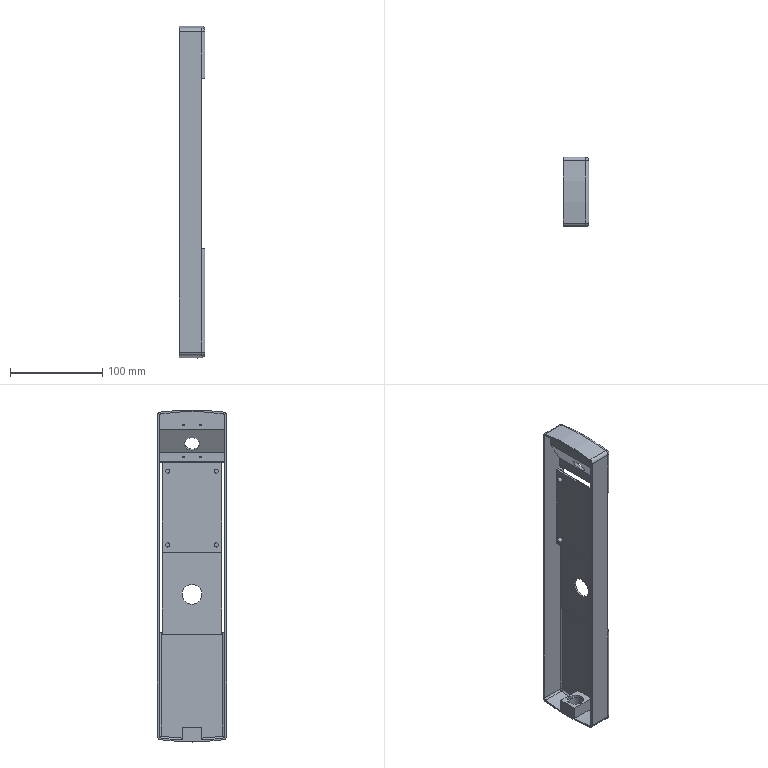Component | NX | TOUCH_HOUSING | 1 solid | 127 faces | volume 107924 mm3 | plane 60 | cylinder 50 | torus 9 | sphere 8 | commonest cylinder face diameters 4 x12 8 x8 1.6 x8 467.75 x4 4.5 x4 6 x4 0.3 x4 471.75 x2